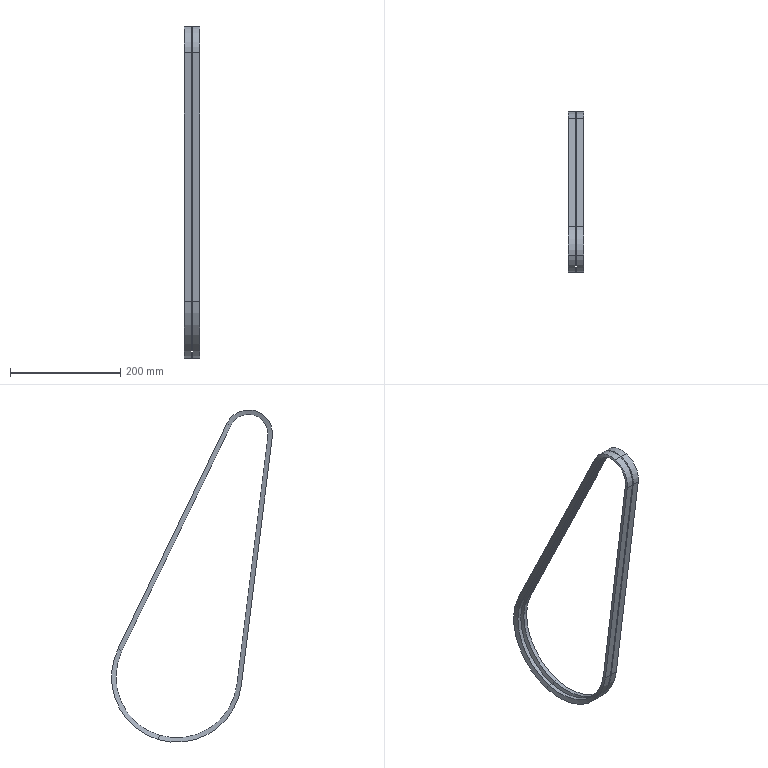Component | SolidWorks | V-beltL459x2-1 | 2 solids | 44 faces | box 28 x 291.38 x 601.58 mm | volume 228297 mm3 | cylinder 16 | plane 16 | cone 12 | commonest cylinder face diameters 219.875 x4 235.875 x4 86.875 x4 70.875 x4 | material Rubber
build123d program:
from build123d import *

# Parameters (mm, degrees)
LPATTERN1_COUNT = 2
LPATTERN1_PITCH = 15


with BuildPart() as part:
    # Sweep1: sweep along a path in Sketch1
    with BuildLine(Plane(origin=(0, 0, 0), x_dir=(0, 0, -1), z_dir=(1, 0, 0))) as sweep1_path:
        Line((19.142, 116.374), (466.05, 42.862))
        ThreePointArc((466.05, 42.862), (502.438, 0), (466.05, -42.862))
        Line((466.05, -42.862), (19.142, -116.374))
        ThreePointArc((19.142, -116.374), (-117.938, 0), (19.142, 116.374))
    # Sketch2 → Sweep1 (sweep)
    with BuildSketch(Plane(origin=(0, 0, 0), x_dir=(1, 0, 0), z_dir=(0, 1, 0))):
        Polygon((-3.588, -109.938), (3.588, -109.938), (6.5, -117.938), (-6.5, -117.938), align=None)
    sweep(path=sweep1_path.line)


with BuildPart() as lpattern1_1:
    # LPattern1: pattern copy
    add(part.part.moved(Location(Vector(1, 0, 0) * (1 * LPATTERN1_PITCH))))


solid = Compound([part.part, lpattern1_1.part])

# Placed as in the assembly
solid = solid.moved(Location((-524.364, 0, 0), (-163.547, 0, -180)))